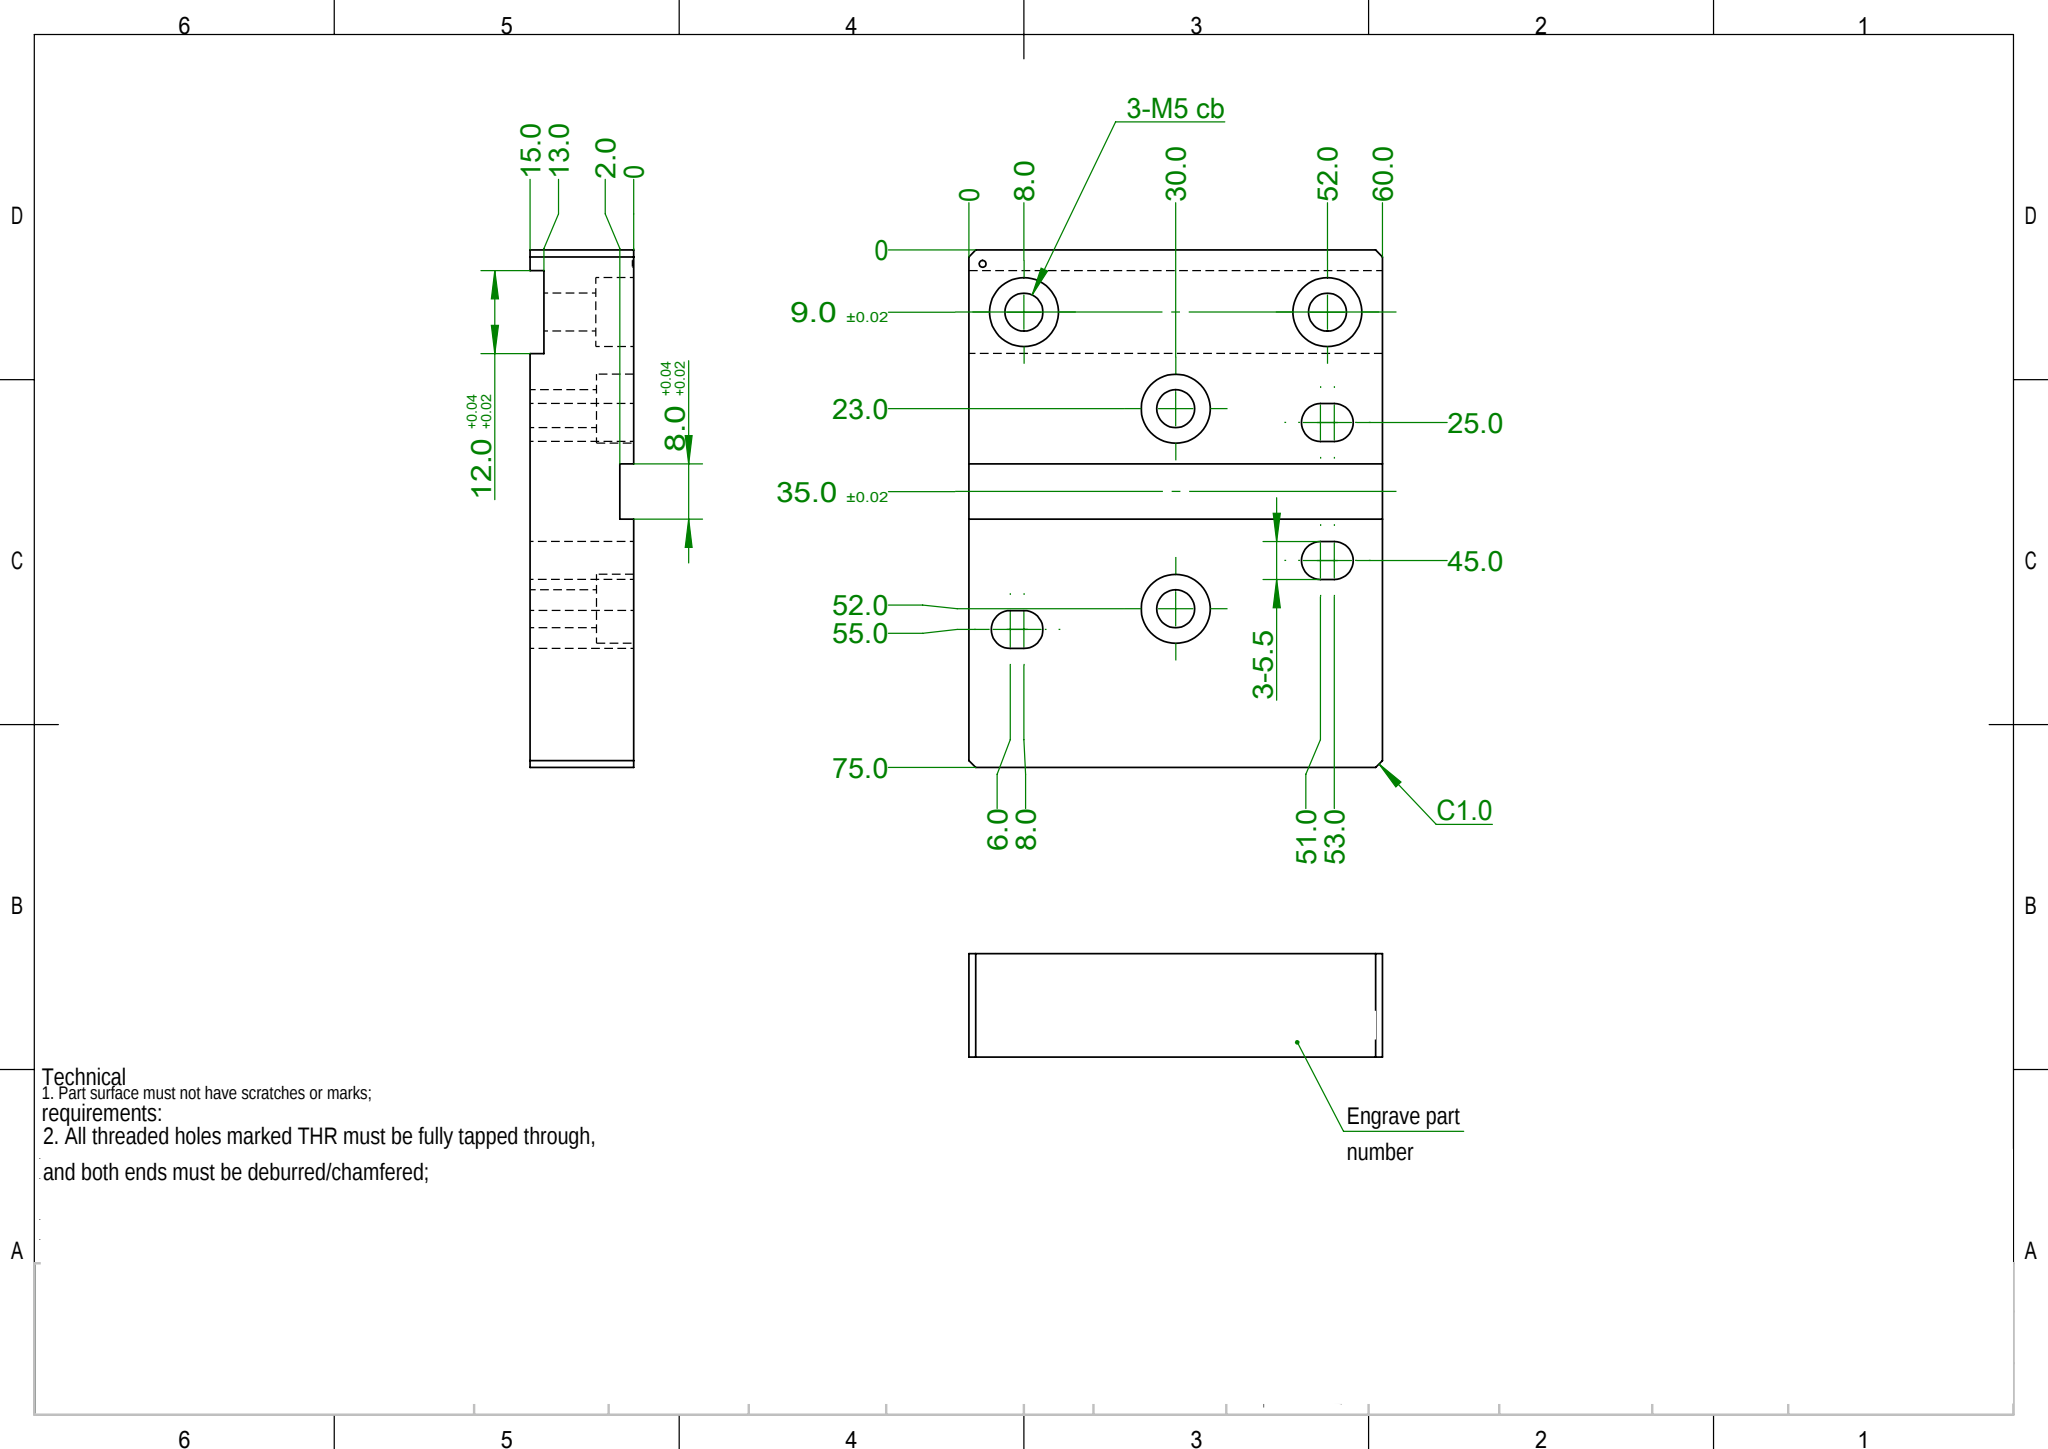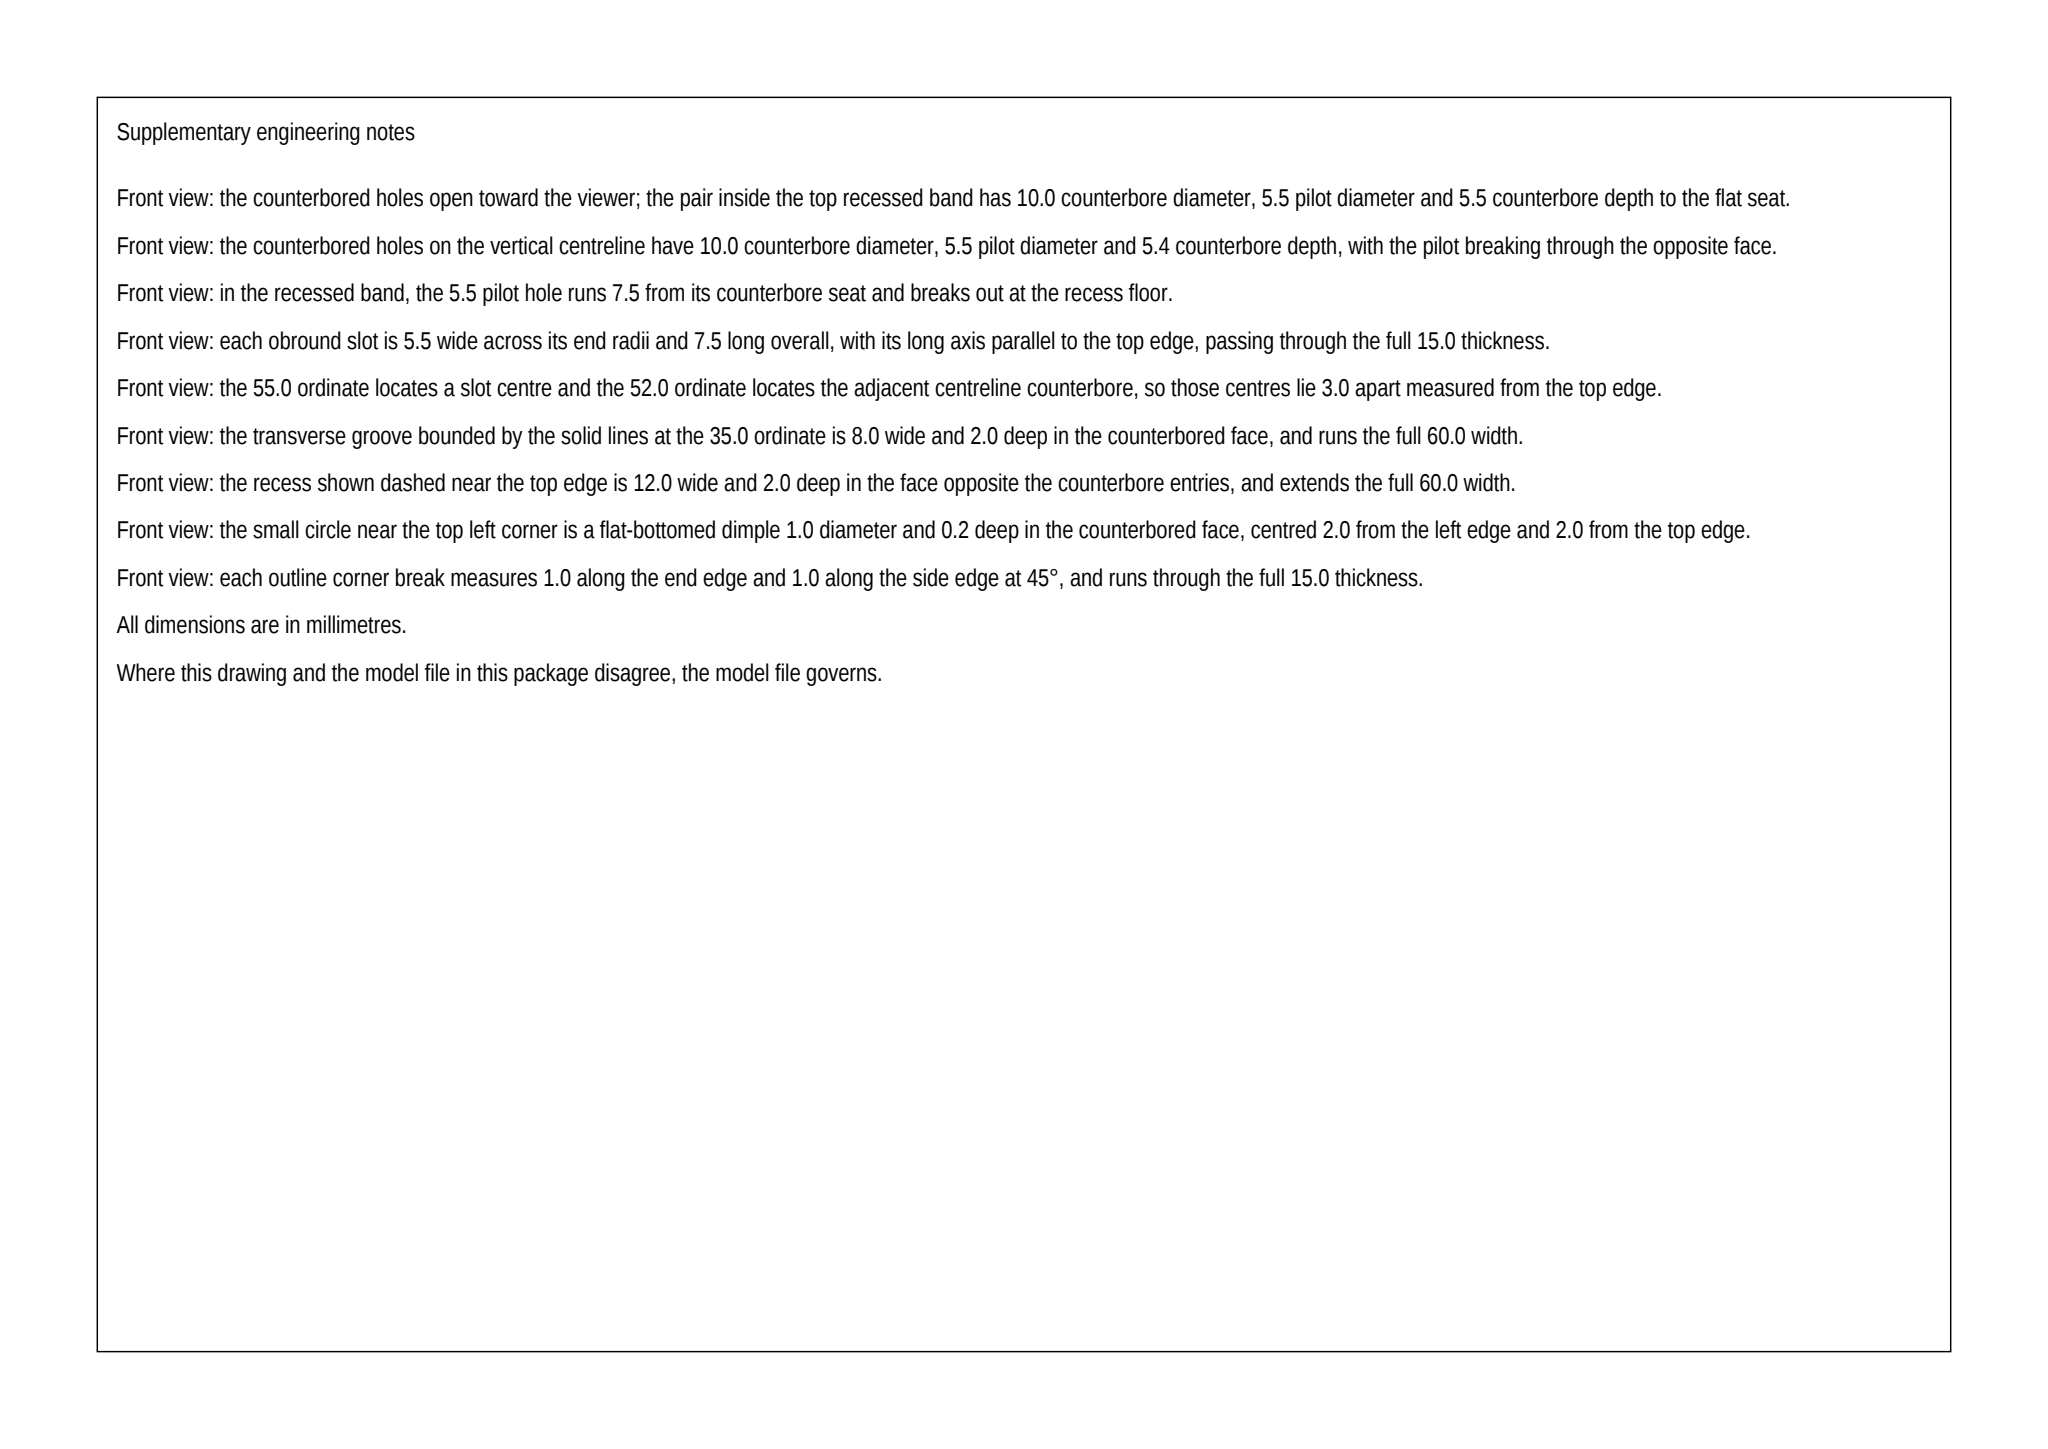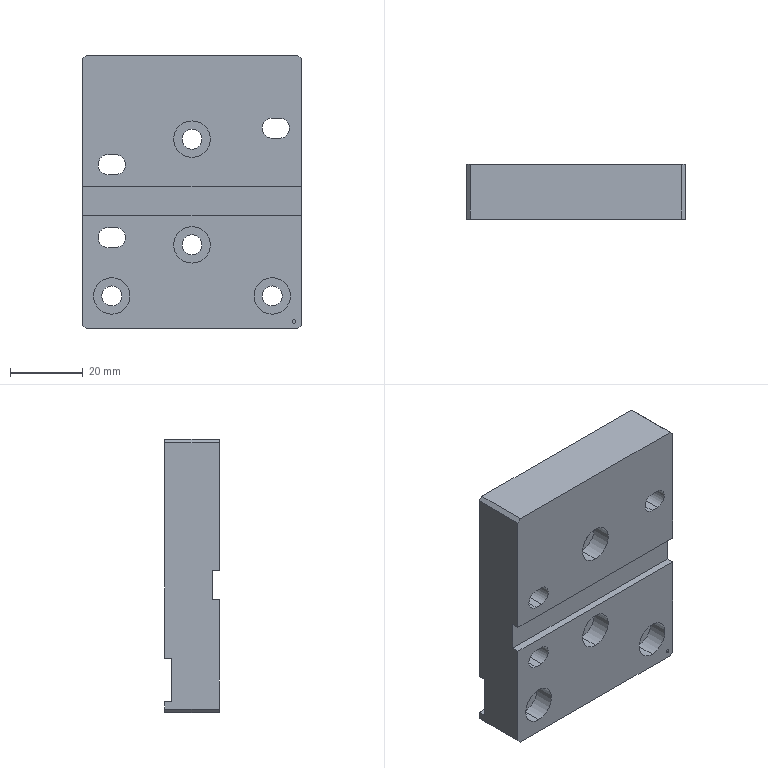Part | SolidWorks | mm | 1 solid | 53 faces | box 60 x 15 x 75 mm | volume 60981 mm3 | plane 29 | cylinder 24 | commonest cylinder face diameters 5.5 x14 10 x8 1 x2
Drawing notes:
BACK FACE STEP 2.0 DP x 12.0 HI: 3.0 FROM TOP EDGE | from the solid: y-planes 2.0 & 13.0 (2.0 deep off 15.0 thk); z-planes 3.0 and 15.0 give 12.0 high step starting 3.0 from top edge (z=0)
3X OBROUND SLOT 5.5 WIDE x 2.0 CTR-TO-CTR, THRU (15.0 THICKNESS): SLOT CENTERS X7.0 & X9.0 AT Z25.0; X7.0 & X9.0 AT Z45.0; X52.0 & X54.0 AT Z55.0 (FROM MIN-CORNER DATUM X0/Z0) | from the solid: cylinders dia 5.5 axis y length 15.0 at (x7,z25),(x9,z25),(x7,z45),(x9,z45),(x52,z55),(x54,z55); bbox y = 15.0
M5 CBORE HOLES ARE 2X ONLY: Ø5.5 THRU, CBORE Ø10.0 DP 5.4 NEAR & FAR FACE, AT X30.0, Z23.0 AND X30.0, Z52.0 (FROM MIN-CORNER DATUM) | from the solid: cylinders [5.5,y,(30,-,23),9.6,2] & [5.5,y,(30,-,52),9.6,2] with [10.0,y,(30,-,23),5.4,2] & [10.0,y,(30,-,52),5.4,2]
Ø5.5 CBORE HOLES ARE 2X ONLY: Ø5.5 THRU, CBORE Ø10.0 DP 5.5 NEAR & FAR FACE, AT X8.0, Z9.0 AND X52.0, Z9.0 (FROM MIN-CORNER DATUM) | from the solid: cylinders [5.5,y,(8,-,9),7.5,2] & [5.5,y,(52,-,9),7.5,2] with [10.0,y,(8,-,9),5.5,2] & [10.0,y,(52,-,9),5.5,2]